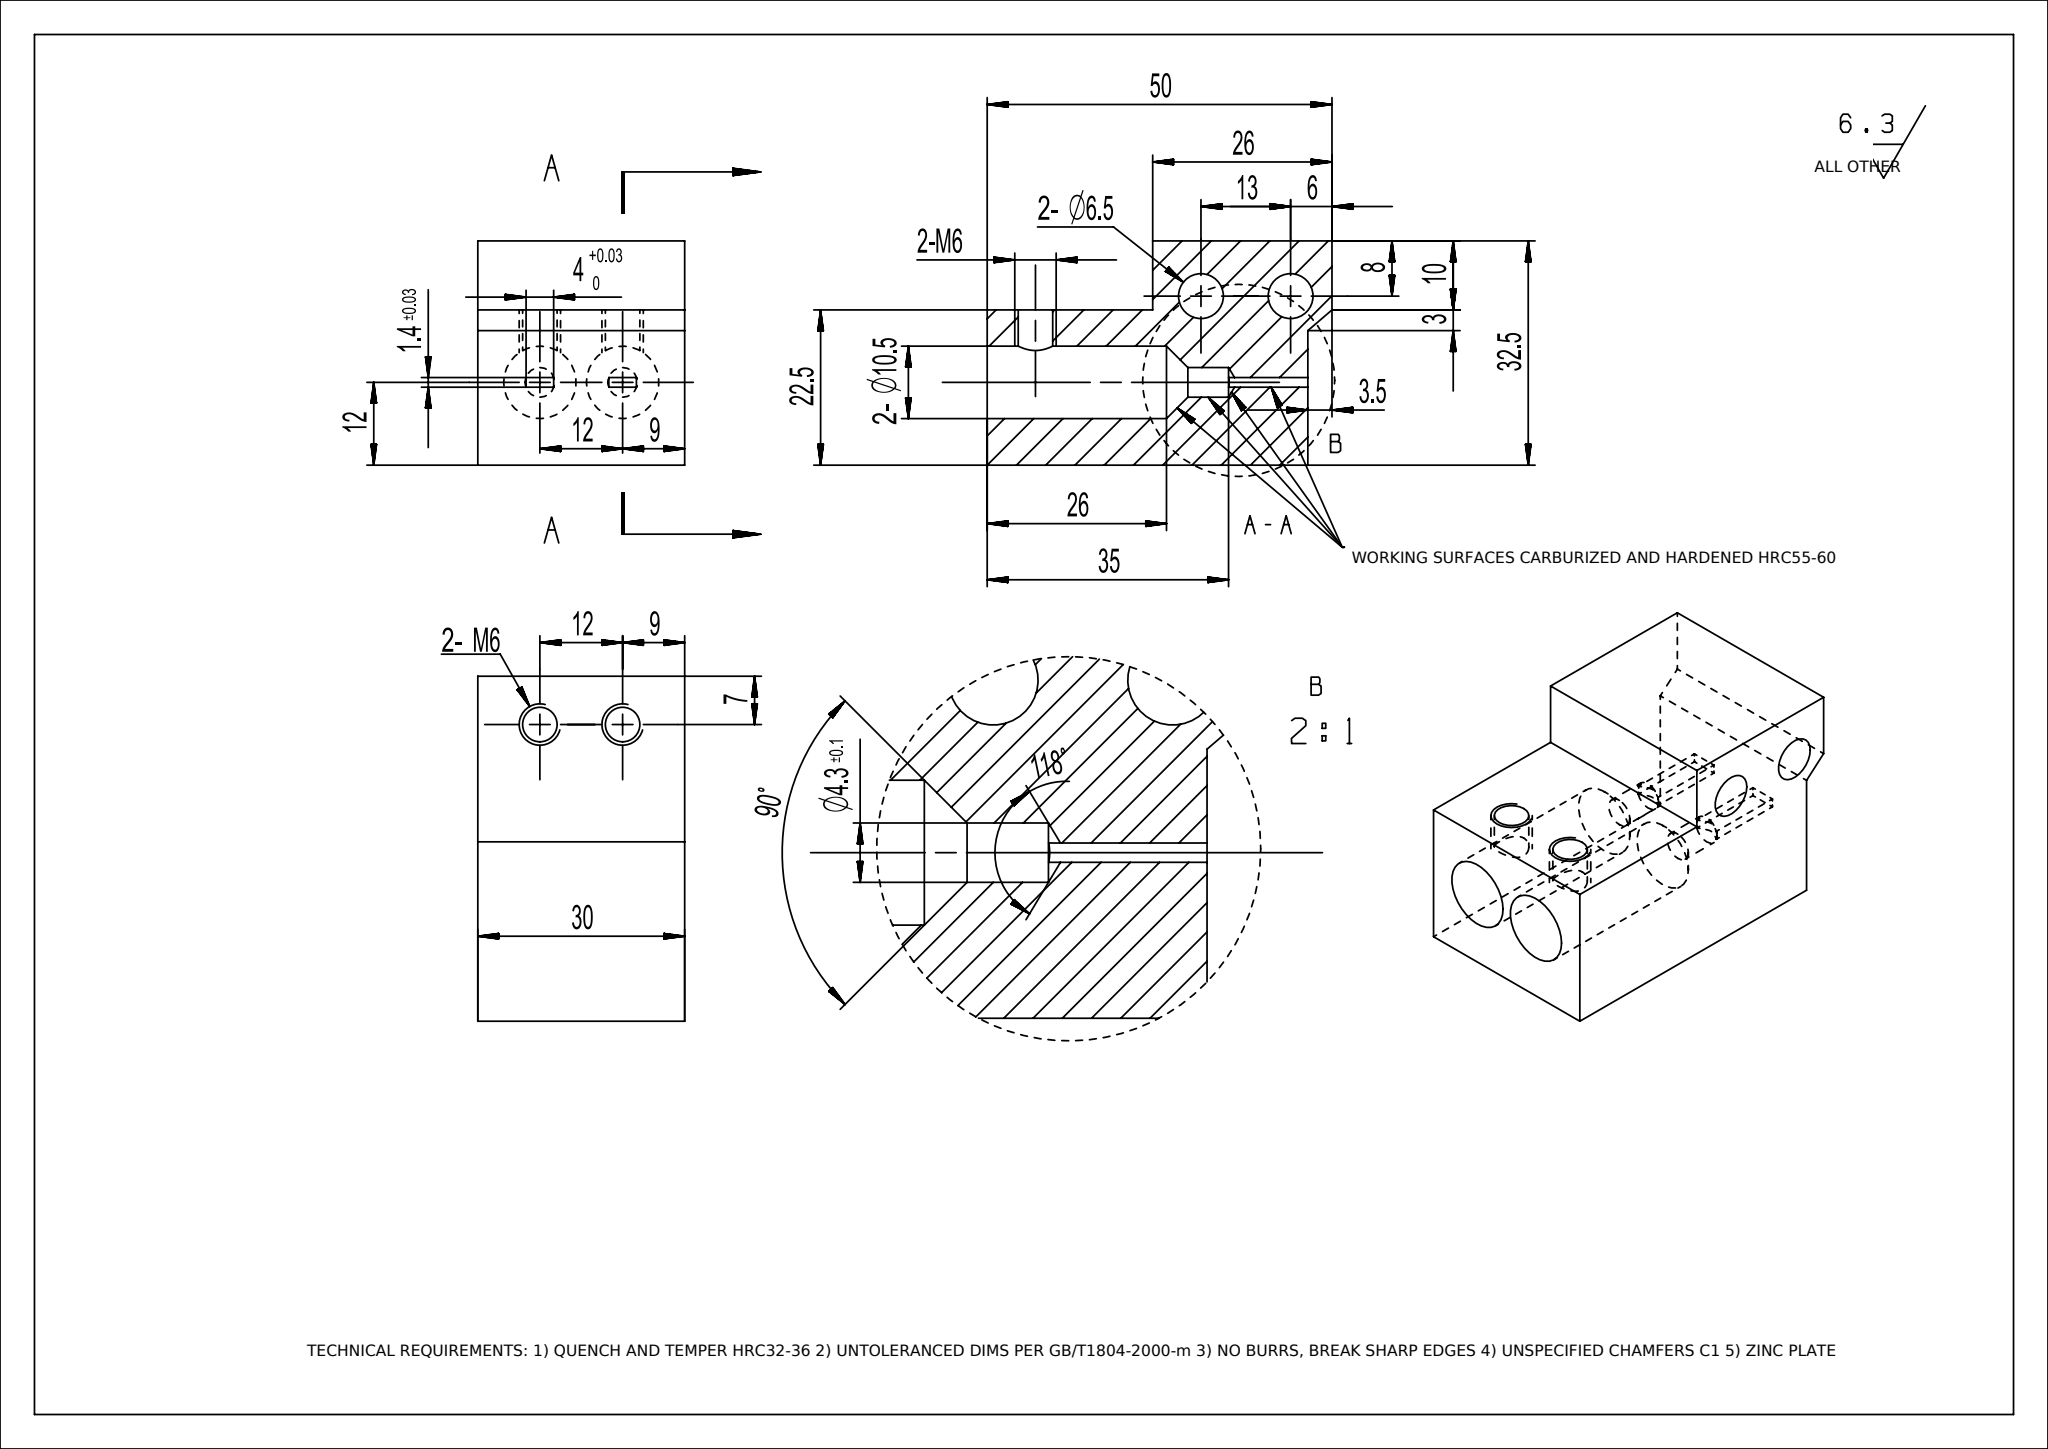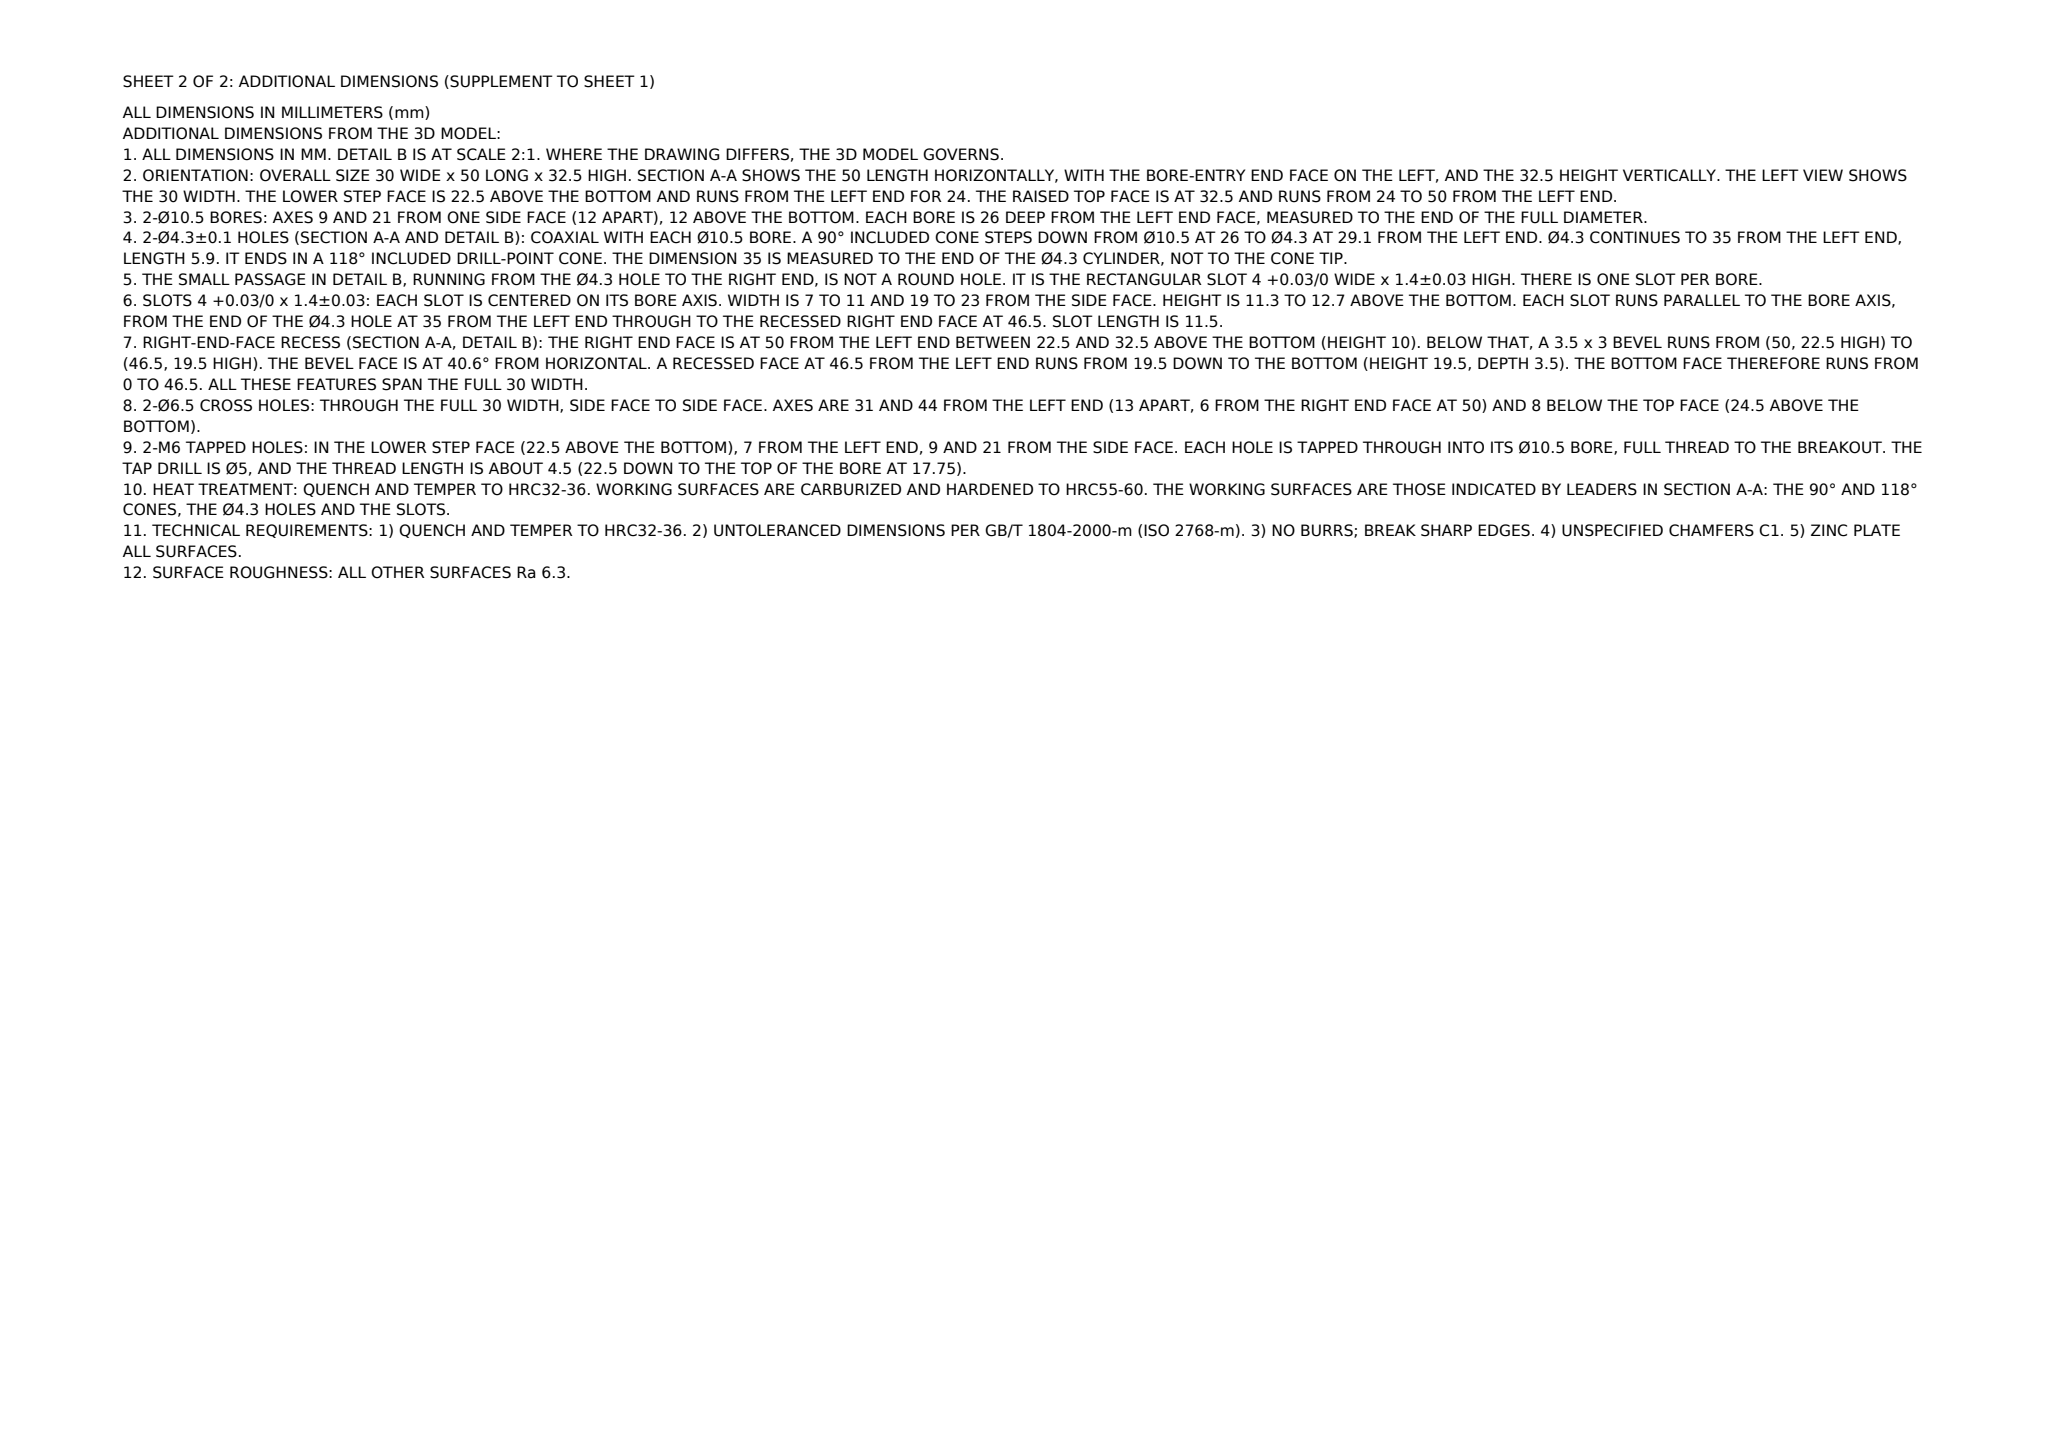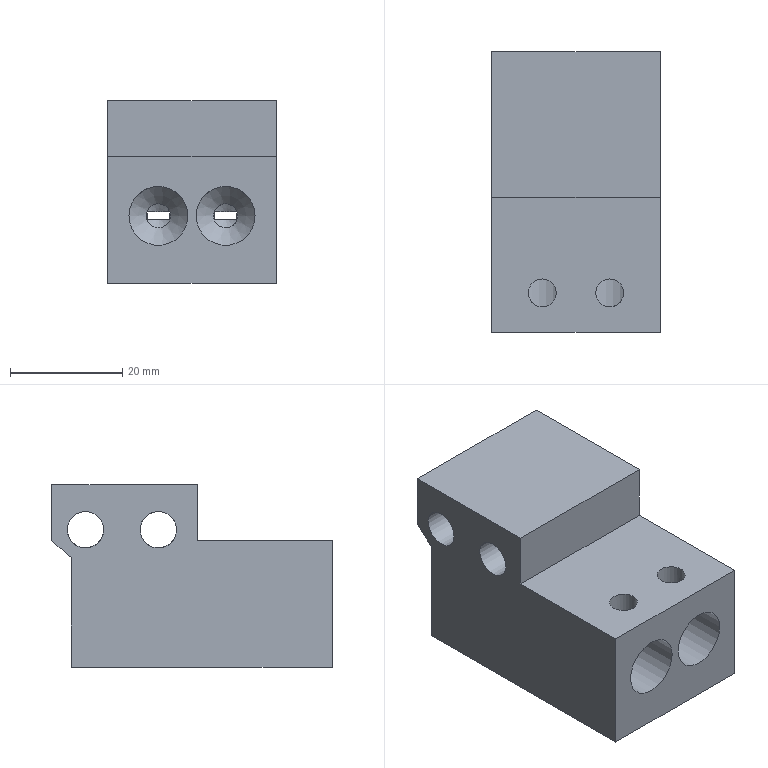Part | NX | mm | 1 solid | 30 faces | box 30 x 50 x 32.5 mm | volume 32051 mm3 | plane 18 | cylinder 8 | cone 4 | commonest cylinder face diameters 6.5 x2 10.5 x2 4.3 x2 5 x2